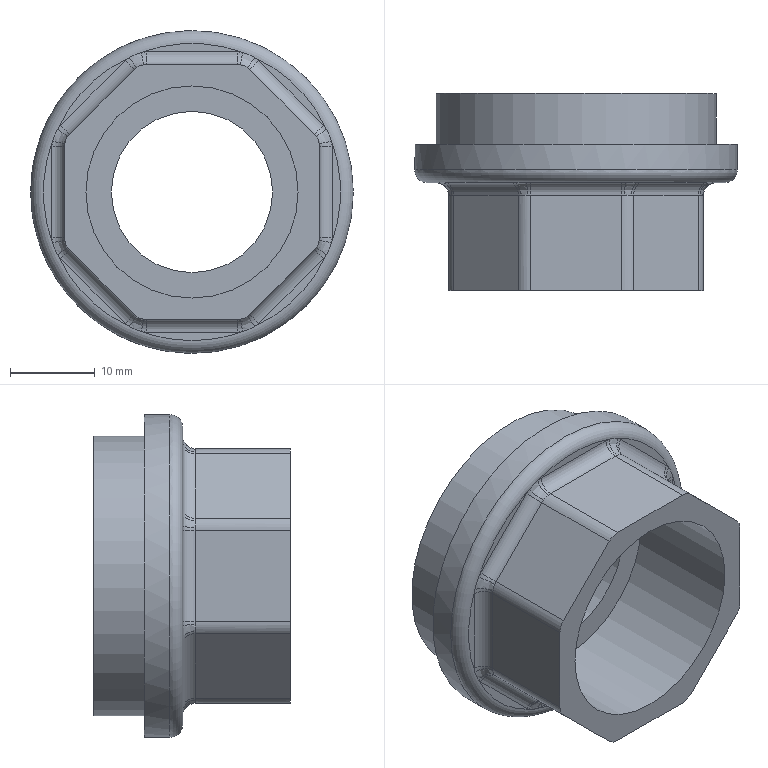Component | NX | VALVE_BONNET | 1 solid | 67 faces | volume 8722 mm3 | plane 21 | cylinder 21 | torus 17 | spline 8 | commonest cylinder face diameters 4 x8 3 x8 19 x1 33 x1 38 x1 26 x1 25 x1